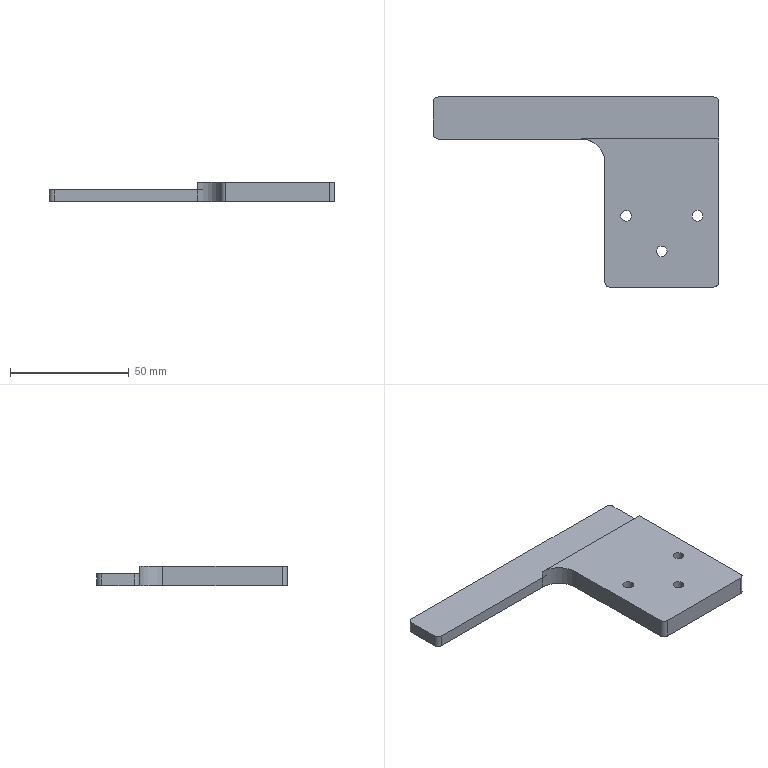CAM job | Mastercam | mm | 9 operations | part box 120 x 80 x 8
1. Drill/Counterbore | 2 - 6定位倒角
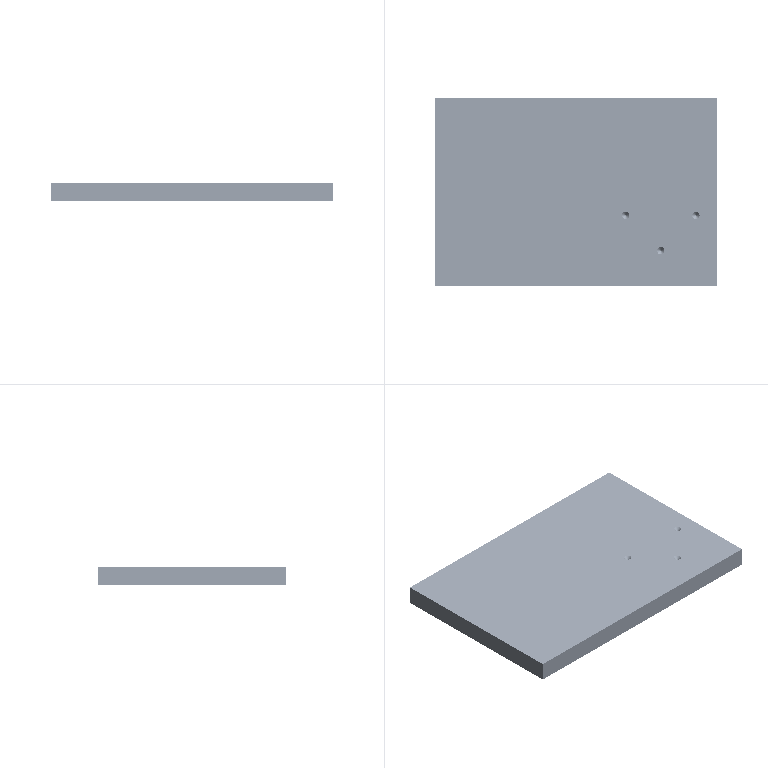2. Peck Drill | 18 - 4.5 钻头
3. Contour (Ramp) | 9 - 10C 平底刀
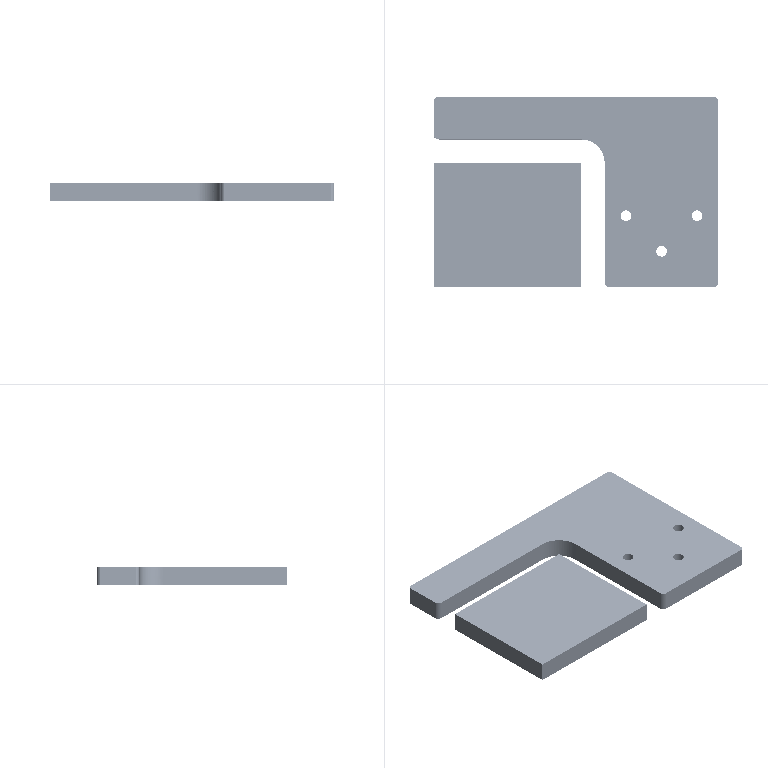4. 2D High Speed (2D Blend Mill) | 3 - 8 C 平底刀
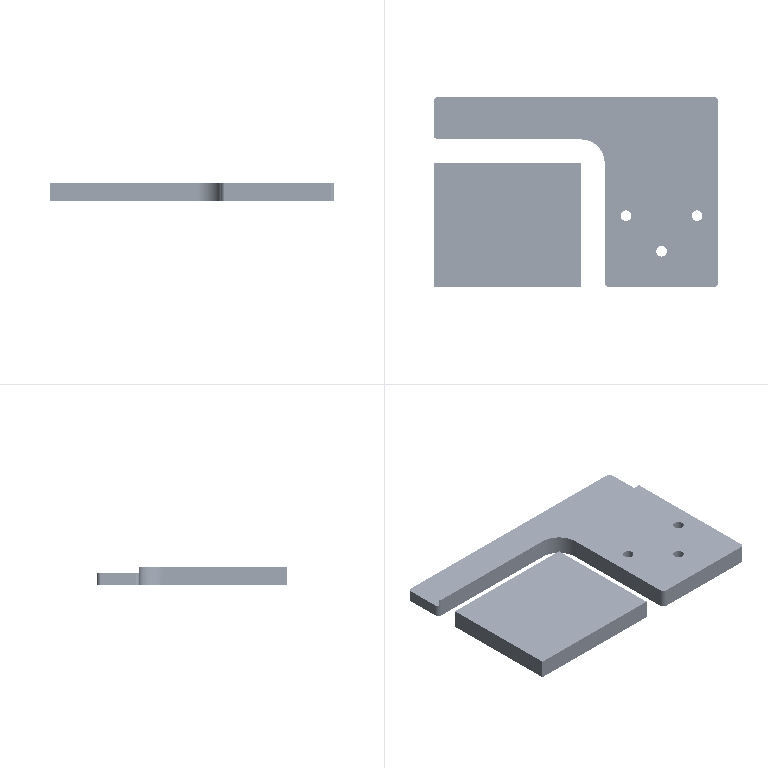5. 2D High Speed (2D Blend Mill) | 4 - 8 J平底刀
6. Contour (2D) | 4 - 8 J平底刀
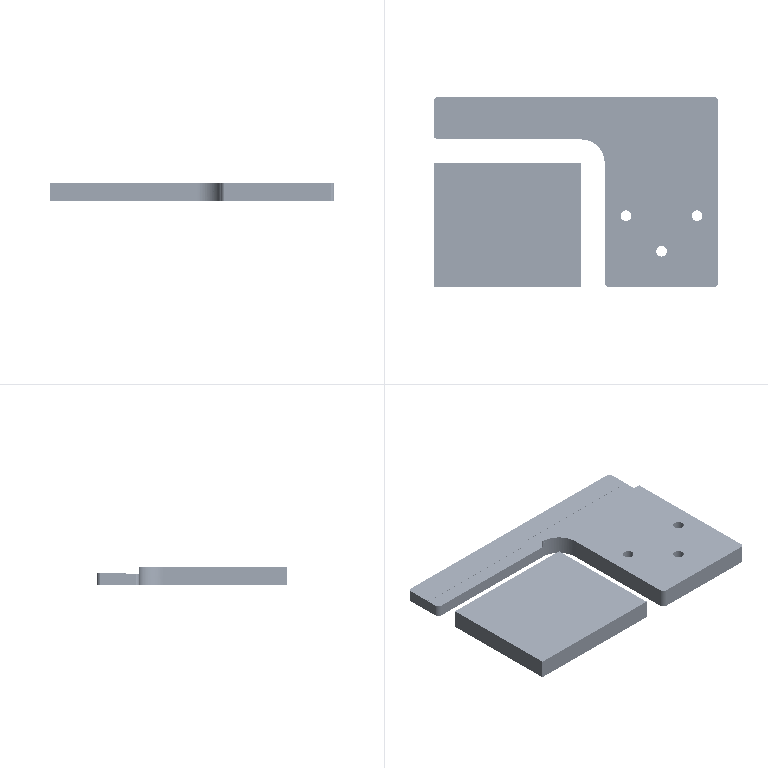7. Contour (2D) | 4 - 8 J平底刀
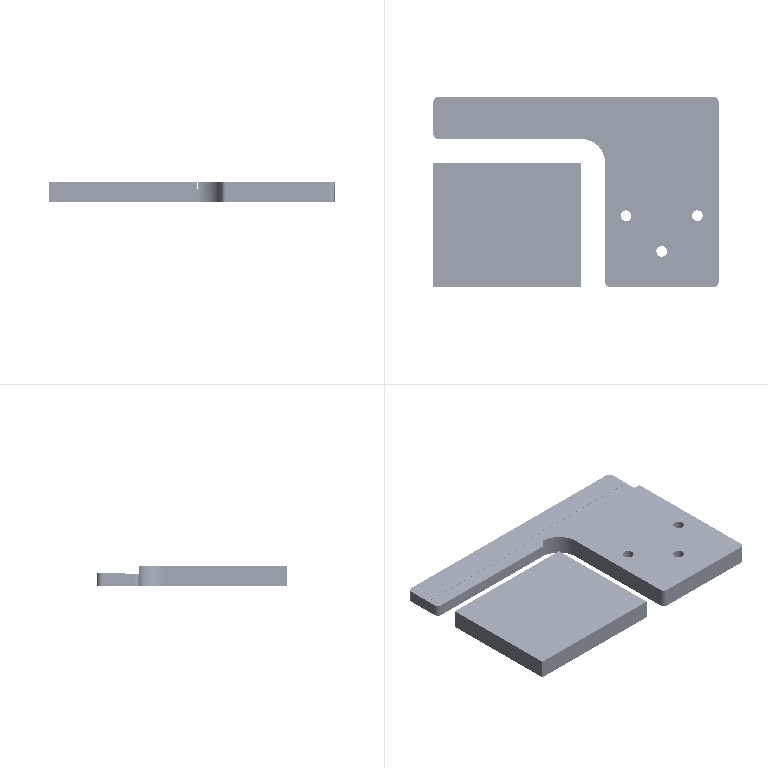8. Model Chamfer | 2 - 6定位倒角
9. Contour (2D) | 4 - 8 J平底刀